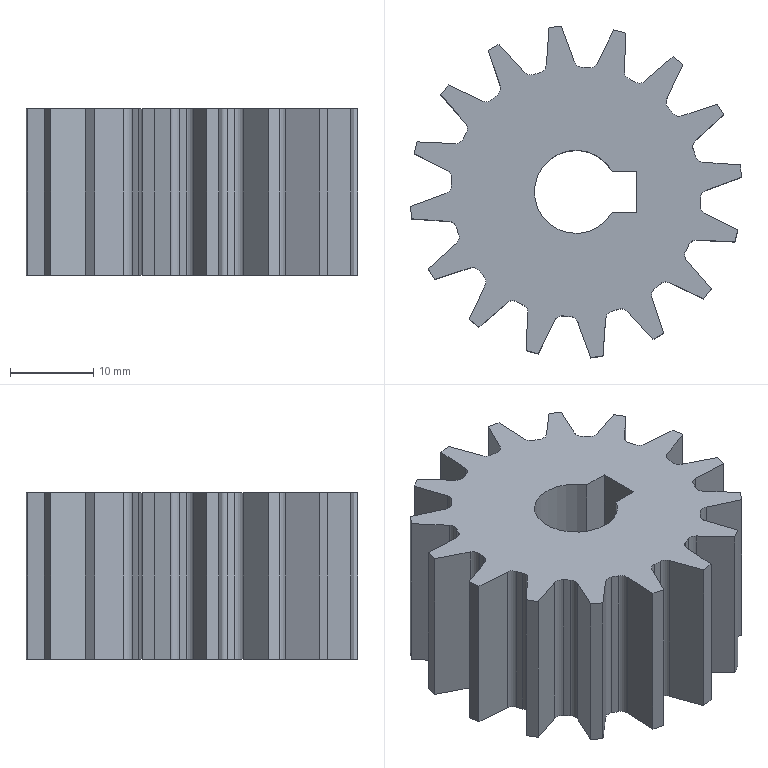Component | SolidWorks | SmallPulley3-1 | 1 solid | 108 faces | box 39.9 x 39.9 x 20 mm | volume 16516 mm3 | cylinder 55 | plane 53 | commonest cylinder face diameters 2 x38 30 x16 10 x1
build123d program:
from build123d import *

# Parameters (mm, degrees)
SKETCH1_2_R              = 15
BOSS_EXTRUDE1_DEPTH      = 20
BOSS_EXTRUDE2_DEPTH      = 20
FILLET1_R                = 1
CIRPATTERN1_COUNT        = 16
FILLET1_OF_CIRPATTERN1_R = 1
SKETCH3_R                = 5
CUT_EXTRUDE1_DEPTH       = 45
REPAIR_KEYWAY5MM_DEPTH   = 50


with BuildPart() as part:
    # Sketch1_2 → Boss-Extrude1 (new body)
    with BuildSketch(Plane.XY):
        Circle(SKETCH1_2_R)
    extrude(amount=BOSS_EXTRUDE1_DEPTH)

    # Sketch2 → Boss-Extrude2 (add)
    with BuildSketch(Plane.XY.offset(20)):
        Polygon((-0.5, 20), (1, 20), (2.094, 14.853), (-1.581, 14.916), align=None)
    boss_extrude2 = extrude(amount=-BOSS_EXTRUDE2_DEPTH)

    # Fillet1
    fillet1_edges = [part.edges().sort_by_distance(p)[0] for p in [
        (2.094, 14.853, 10),
        (-1.581, 14.916, 10),
    ]]
    fillet(fillet1_edges, radius=FILLET1_R)

    # CirPattern1: Boss-Extrude2 ×16 about axis
    cirpattern1_axis = Axis((0, 0, 0), (0, 0, 1))
    for i in range(1, CIRPATTERN1_COUNT):
        add(boss_extrude2.rotate(cirpattern1_axis, i * 360 / CIRPATTERN1_COUNT))

    # Fillet1 of CirPattern1
    fillet1_of_cirpattern1_edges = [part.edges().sort_by_distance(p)[0] for p in [
        (-3.749, 14.524, 10),
        (-7.169, 13.176, 10),
        (-9.022, 11.983, 10),
        (-11.665, 9.43, 10),
        (-12.921, 7.619, 10),
        (-14.386, 4.248, 10),
        (-14.853, 2.094, 10),
        (-14.916, -1.581, 10),
        (-14.524, -3.749, 10),
        (-13.176, -7.169, 10),
        (-11.983, -9.022, 10),
        (-9.43, -11.665, 10),
        (-7.619, -12.921, 10),
        (-4.248, -14.386, 10),
        (-2.094, -14.853, 10),
        (1.581, -14.916, 10),
        (3.749, -14.524, 10),
        (7.169, -13.176, 10),
        (9.022, -11.983, 10),
        (11.665, -9.43, 10),
        (12.921, -7.619, 10),
        (14.386, -4.248, 10),
        (14.853, -2.094, 10),
        (14.916, 1.581, 10),
        (14.524, 3.749, 10),
        (13.176, 7.169, 10),
        (11.983, 9.022, 10),
        (9.43, 11.665, 10),
        (7.619, 12.921, 10),
        (4.248, 14.386, 10),
    ]]
    fillet(fillet1_of_cirpattern1_edges, radius=FILLET1_OF_CIRPATTERN1_R)

    # Sketch3 → Cut-Extrude1 (cut)
    with BuildSketch(Plane.XY.offset(20)):
        Circle(SKETCH3_R)
    extrude(amount=-CUT_EXTRUDE1_DEPTH, mode=Mode.SUBTRACT)

    # Sketch1 → Repair_Keyway5mm (cut, symmetric)
    with BuildSketch(Plane.XY):
        Polygon((2.628, -2.888), (6.888, -3.479), (7.574, 1.474), (3.315, 2.064), align=None)
    extrude(amount=REPAIR_KEYWAY5MM_DEPTH, both=True, mode=Mode.SUBTRACT)


solid = part.part

# Placed as in the assembly
solid = solid.moved(Location((246.241, -267.715, 1435.724), (0, 0, 7.892)))